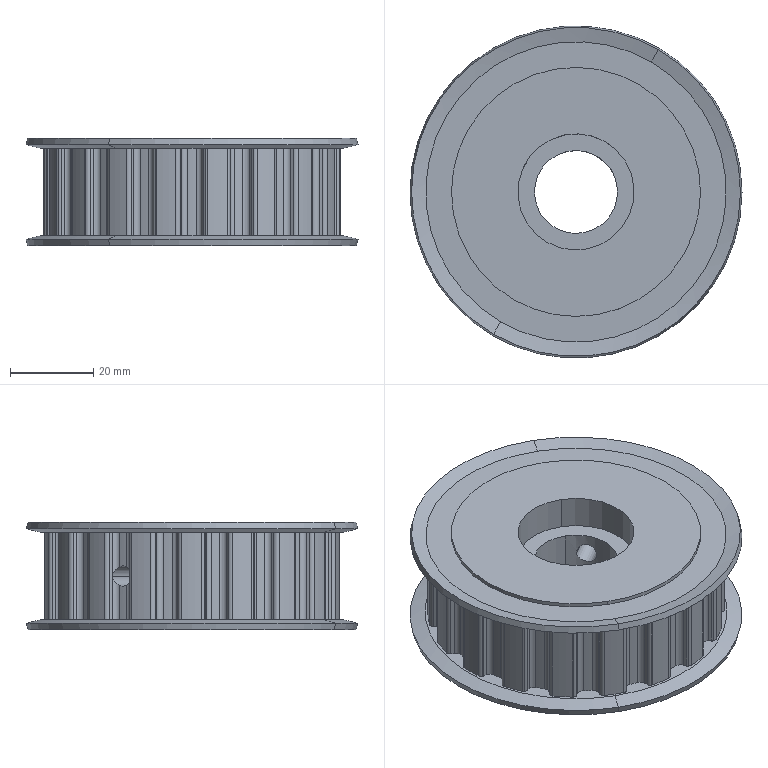Component | SolidWorks | ATPA18H075-1 | 1 solid | 195 faces | volume 86349 mm3 | cylinder 138 | plane 45 | cone 12 | commonest cylinder face diameters 2.94 x43 2.08 x42 66.21 x20 71.39 x19 28 x4 60 x4 4.917 x4 20 x2